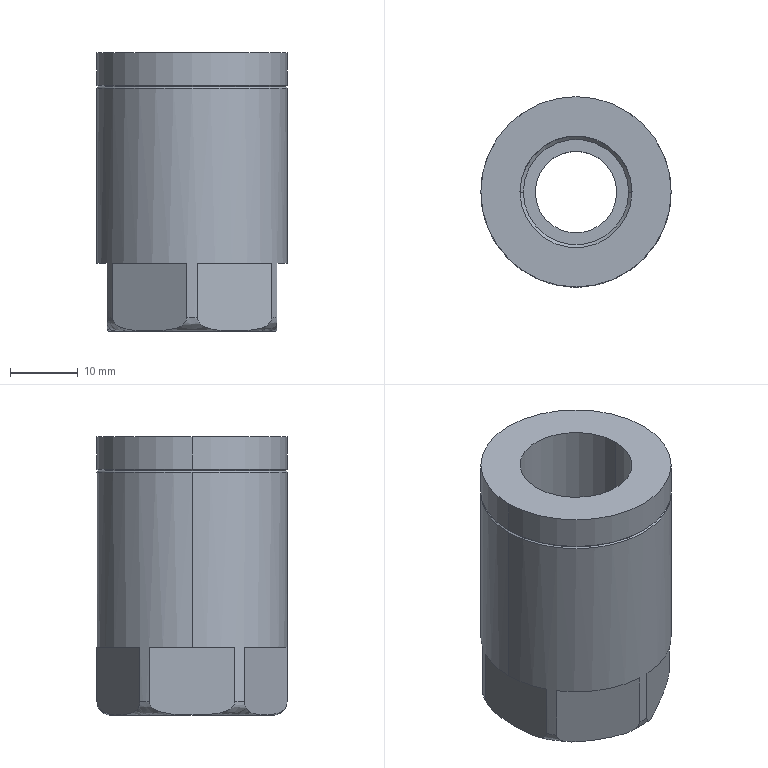Component | SolidWorks | JDAD32x50-20-SE2-1_TIAO-1 | 1 solid | 31 faces | volume 16806 mm3 | plane 15 | cylinder 8 | cone 6 | spline 2 | commonest cylinder face diameters 28 x4 12 x2 16.5 x2